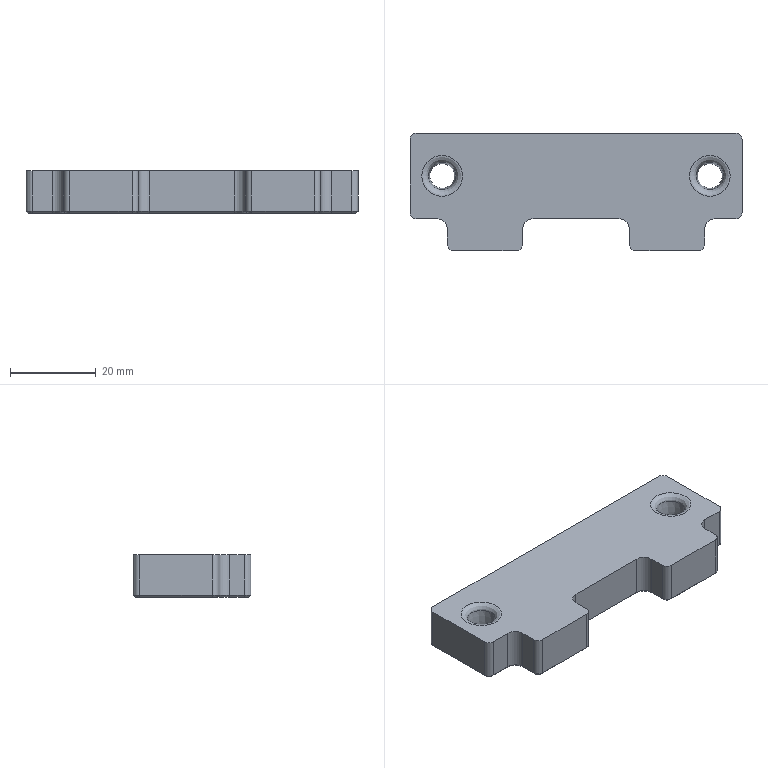Component | NX | JIAZHONGKUAI | 1 solid | 56 faces | volume 17491 mm3 | plane 26 | cone 16 | cylinder 12 | torus 2 | commonest cylinder face diameters 3 x8 5 x4